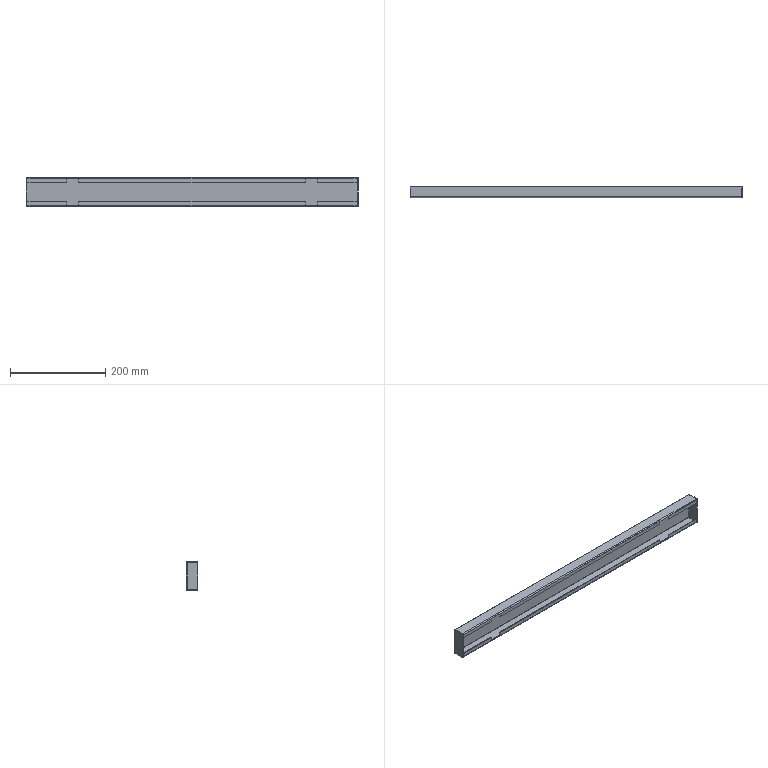Component | SolidWorks | Brow-1 | 1 solid | 82 faces | volume 129155 mm3 | plane 70 | cylinder 12 | commonest cylinder face diameters 4 x6 1 x6